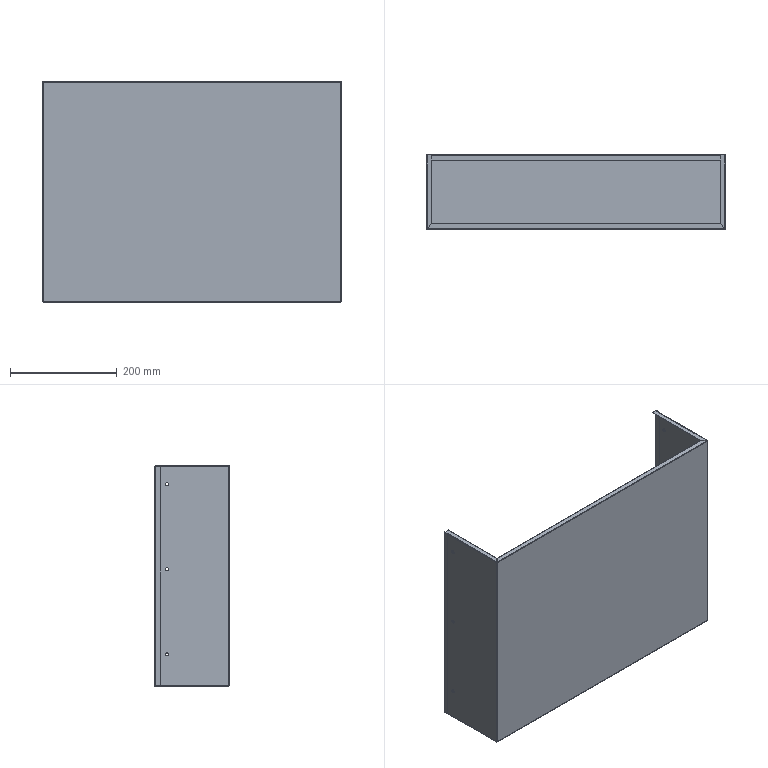Component | SolidWorks | PC-CAJ-P08-1_PC-CAJ-P18-1_PM-CAJ-P58-1 | 1 solid | 99 faces | volume 311807 mm3 | plane 62 | cylinder 33 | spline 4 | commonest cylinder face diameters 6 x12 1 x6 2.4 x6 1.6 x5 0.2 x4 | material Plain Carbon Steel